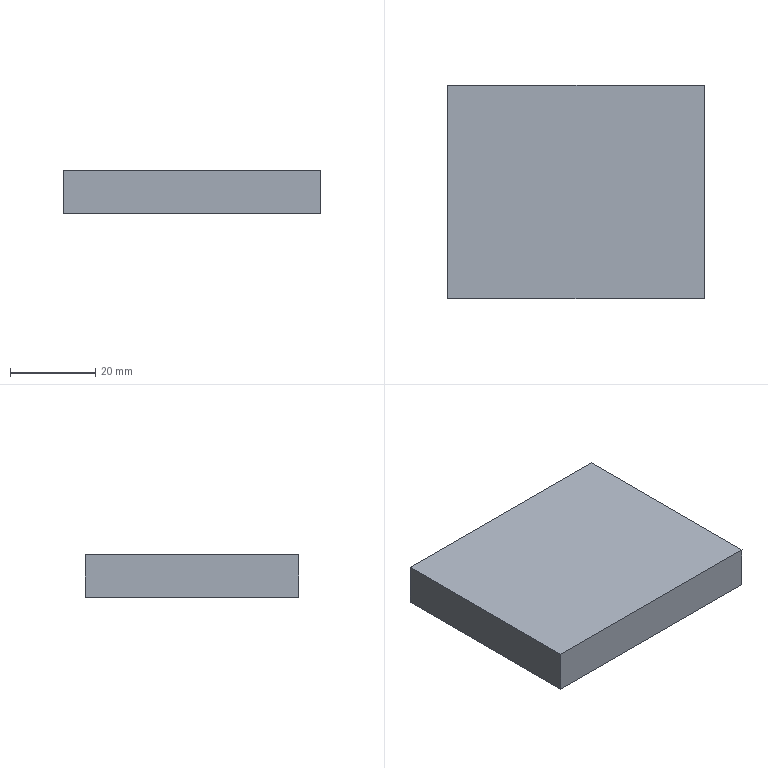Component | SolidWorks | 02-1 | 1 solid | 12 faces | box 60 x 50 x 10 mm | volume 29478 mm3 | plane 8 | cylinder 4 | commonest cylinder face diameters 6.5 x2 5 x2
build123d program:
from build123d import *

# Parameters (mm, degrees)
SKETCH1_2_W               = 60
SKETCH1_2_H               = 50
BOSS_EXTRUDE1_DEPTH       = 5
SKETCH1_R                 = 2.5
M5_TAP_CDJ2B_RODEND_DEPTH = 8
SKETCH2_R                 = 3.25
BUFFER_STOP_POCKET_DEPTH  = 11


with BuildPart() as part:
    # Sketch1_2 → Boss-Extrude1 (new, symmetric)
    with BuildSketch(Plane.XY):
        Rectangle(SKETCH1_2_W, SKETCH1_2_H)
    extrude(amount=BOSS_EXTRUDE1_DEPTH, both=True)

    # Sketch1 → M5_Tap_CDJ2B_RodEnd (cut)
    with BuildSketch(Plane.ZY.offset(30)):
        with Locations((0, -13.3)):
            Circle(SKETCH1_R)
    extrude(amount=-M5_TAP_CDJ2B_RODEND_DEPTH, mode=Mode.SUBTRACT)

    # Sketch2 → Buffer_Stop_Pocket (cut)
    with BuildSketch(Plane.ZY.offset(30)):
        with Locations((0, 11.7)):
            Circle(SKETCH2_R)
    extrude(amount=-BUFFER_STOP_POCKET_DEPTH, mode=Mode.SUBTRACT)


solid = part.part

# Placed as in the assembly
solid = solid.moved(Location((-42, 208.3, 39), (-180, 0, 180)))
STEP:
#1=CARTESIAN_POINT('',(-0.9055,8.661,1.663));
#2=VERTEX_POINT('',#1);
#3=CARTESIAN_POINT('',(-0.9055,8.661,1.407));
#4=VERTEX_POINT('',#3);
#5=CARTESIAN_POINT('',(-0.9055,8.661,1.535));
#6=DIRECTION('',(1.,0.,-0.));
#7=DIRECTION('',(0.,0.,-1.));
#8=AXIS2_PLACEMENT_3D('',#5,#6,#7);
#9=CIRCLE('',#8,0.128);
#10=EDGE_CURVE('',#2,#4,#9,.T.);
#11=ORIENTED_EDGE('',*,*,#10,.F.);
#12=CARTESIAN_POINT('',(-0.4724,8.661,1.663));
#13=VERTEX_POINT('',#12);
#14=CARTESIAN_POINT('',(-0.9055,8.661,1.663));
#15=DIRECTION('',(1.,0.,-0.));
#16=VECTOR('',#15,39.37);
#17=LINE('',#14,#16);
#18=EDGE_CURVE('',#2,#13,#17,.T.);
#19=ORIENTED_EDGE('',*,*,#18,.T.);
#20=CARTESIAN_POINT('',(-0.4724,8.661,1.407));
#21=VERTEX_POINT('',#20);
#22=CARTESIAN_POINT('',(-0.4724,8.661,1.535));
#23=DIRECTION('',(1.,0.,-0.));
#24=DIRECTION('',(0.,0.,-1.));
#25=AXIS2_PLACEMENT_3D('',#22,#23,#24);
#26=CIRCLE('',#25,0.128);
#27=EDGE_CURVE('',#13,#21,#26,.T.);
#28=ORIENTED_EDGE('',*,*,#27,.T.);
#29=CARTESIAN_POINT('',(-0.9055,8.661,1.407));
#30=DIRECTION('',(1.,0.,-0.));
#31=VECTOR('',#30,39.37);
#32=LINE('',#29,#31);
#33=EDGE_CURVE('',#4,#21,#32,.T.);
#34=ORIENTED_EDGE('',*,*,#33,.F.);
#35=EDGE_LOOP('',(#11,#19,#28,#34));
#36=FACE_OUTER_BOUND('',#35,.T.);
#37=CARTESIAN_POINT('',(-0.9055,8.661,1.535));
#38=DIRECTION('',(1.,0.,-0.));
#39=DIRECTION('',(0.,0.,-1.));
#40=AXIS2_PLACEMENT_3D('',#37,#38,#39);
#41=CYLINDRICAL_SURFACE('',#40,0.128);
#42=ADVANCED_FACE('',(#36),#41,.F.);
#43=CARTESIAN_POINT('',(-0.7874,7.677,1.634));
#44=VERTEX_POINT('',#43);
#45=CARTESIAN_POINT('',(-0.7874,7.677,1.437));
#46=VERTEX_POINT('',#45);
#47=CARTESIAN_POINT('',(-0.7874,7.677,1.535));
#48=DIRECTION('',(1.,0.,-0.));
#49=DIRECTION('',(0.,0.,-1.));
#50=AXIS2_PLACEMENT_3D('',#47,#48,#49);
#51=CIRCLE('',#50,0.09843);
#52=EDGE_CURVE('',#44,#46,#51,.T.);
#53=ORIENTED_EDGE('',*,*,#52,.F.);
#54=CARTESIAN_POINT('',(-0.4724,7.677,1.634));
#55=VERTEX_POINT('',#54);
#56=CARTESIAN_POINT('',(-0.7874,7.677,1.634));
#57=DIRECTION('',(1.,0.,-0.));
#58=VECTOR('',#57,39.37);
#59=LINE('',#56,#58);
#60=EDGE_CURVE('',#44,#55,#59,.T.);
#61=ORIENTED_EDGE('',*,*,#60,.T.);
#62=CARTESIAN_POINT('',(-0.4724,7.677,1.437));
#63=VERTEX_POINT('',#62);
#64=CARTESIAN_POINT('',(-0.4724,7.677,1.535));
#65=DIRECTION('',(1.,0.,-0.));
#66=DIRECTION('',(0.,0.,-1.));
#67=AXIS2_PLACEMENT_3D('',#64,#65,#66);
#68=CIRCLE('',#67,0.09843);
#69=EDGE_CURVE('',#55,#63,#68,.T.);
#70=ORIENTED_EDGE('',*,*,#69,.T.);
#71=CARTESIAN_POINT('',(-0.7874,7.677,1.437));
#72=DIRECTION('',(1.,0.,-0.));
#73=VECTOR('',#72,39.37);
#74=LINE('',#71,#73);
#75=EDGE_CURVE('',#46,#63,#74,.T.);
#76=ORIENTED_EDGE('',*,*,#75,.F.);
#77=EDGE_LOOP('',(#53,#61,#70,#76));
#78=FACE_OUTER_BOUND('',#77,.T.);
#79=CARTESIAN_POINT('',(-0.7874,7.677,1.535));
#80=DIRECTION('',(1.,0.,-0.));
#81=DIRECTION('',(0.,0.,-1.));
#82=AXIS2_PLACEMENT_3D('',#79,#80,#81);
#83=CYLINDRICAL_SURFACE('',#82,0.09843);
#84=ADVANCED_FACE('',(#78),#83,.F.);
#85=CARTESIAN_POINT('',(-2.835,7.217,1.732));
#86=VERTEX_POINT('',#85);
#87=CARTESIAN_POINT('',(-2.835,9.185,1.732));
#88=VERTEX_POINT('',#87);
#89=CARTESIAN_POINT('',(-2.835,7.217,1.732));
#90=DIRECTION('',(-0.,1.,0.));
#91=VECTOR('',#90,39.37);
#92=LINE('',#89,#91);
#93=EDGE_CURVE('',#86,#88,#92,.T.);
#94=ORIENTED_EDGE('',*,*,#93,.T.);
#95=CARTESIAN_POINT('',(-2.835,9.185,1.339));
#96=VERTEX_POINT('',#95);
#97=CARTESIAN_POINT('',(-2.835,9.185,1.339));
#98=DIRECTION('',(0.,-0.,1.));
#99=VECTOR('',#98,39.37);
#100=LINE('',#97,#99);
#101=EDGE_CURVE('',#96,#88,#100,.T.);
#102=ORIENTED_EDGE('',*,*,#101,.F.);
#103=CARTESIAN_POINT('',(-2.835,7.217,1.339));
#104=VERTEX_POINT('',#103);
#105=CARTESIAN_POINT('',(-2.835,7.217,1.339));
#106=DIRECTION('',(-0.,1.,0.));
#107=VECTOR('',#106,39.37);
#108=LINE('',#105,#107);
#109=EDGE_CURVE('',#104,#96,#108,.T.);
#110=ORIENTED_EDGE('',*,*,#109,.F.);
#111=CARTESIAN_POINT('',(-2.835,7.217,1.339));
#112=DIRECTION('',(0.,-0.,1.));
#113=VECTOR('',#112,39.37);
#114=LINE('',#111,#113);
#115=EDGE_CURVE('',#104,#86,#114,.T.);
#116=ORIENTED_EDGE('',*,*,#115,.T.);
#117=EDGE_LOOP('',(#94,#102,#110,#116));
#118=FACE_OUTER_BOUND('',#117,.T.);
#119=CARTESIAN_POINT('',(-2.835,7.217,1.339));
#120=DIRECTION('',(1.,0.,-0.));
#121=DIRECTION('',(-0.,0.,-1.));
#122=AXIS2_PLACEMENT_3D('',#119,#120,#121);
#123=PLANE('',#122);
#124=ADVANCED_FACE('',(#118),#123,.F.);
#125=CARTESIAN_POINT('',(-0.4724,9.185,1.732));
#126=VERTEX_POINT('',#125);
#127=CARTESIAN_POINT('',(-0.4724,9.185,1.732));
#128=DIRECTION('',(1.,0.,-0.));
#129=VECTOR('',#128,39.37);
#130=LINE('',#127,#129);
#131=EDGE_CURVE('',#88,#126,#130,.T.);
#132=ORIENTED_EDGE('',*,*,#131,.T.);
#133=CARTESIAN_POINT('',(-0.4724,9.185,1.339));
#134=VERTEX_POINT('',#133);
#135=CARTESIAN_POINT('',(-0.4724,9.185,1.339));
#136=DIRECTION('',(0.,-0.,1.));
#137=VECTOR('',#136,39.37);
#138=LINE('',#135,#137);
#139=EDGE_CURVE('',#134,#126,#138,.T.);
#140=ORIENTED_EDGE('',*,*,#139,.F.);
#141=CARTESIAN_POINT('',(-0.4724,9.185,1.339));
#142=DIRECTION('',(1.,0.,-0.));
#143=VECTOR('',#142,39.37);
#144=LINE('',#141,#143);
#145=EDGE_CURVE('',#96,#134,#144,.T.);
#146=ORIENTED_EDGE('',*,*,#145,.F.);
#147=ORIENTED_EDGE('',*,*,#101,.T.);
#148=EDGE_LOOP('',(#132,#140,#146,#147));
#149=FACE_OUTER_BOUND('',#148,.T.);
#150=CARTESIAN_POINT('',(-0.4724,9.185,1.339));
#151=DIRECTION('',(0.,-1.,-0.));
#152=DIRECTION('',(0.,-0.,1.));
#153=AXIS2_PLACEMENT_3D('',#150,#151,#152);
#154=PLANE('',#153);
#155=ADVANCED_FACE('',(#149),#154,.F.);
#156=CARTESIAN_POINT('',(-0.4724,8.661,1.535));
#157=DIRECTION('',(1.,0.,-0.));
#158=DIRECTION('',(0.,0.,-1.));
#159=AXIS2_PLACEMENT_3D('',#156,#157,#158);
#160=CIRCLE('',#159,0.128);
#161=EDGE_CURVE('',#21,#13,#160,.T.);
#162=ORIENTED_EDGE('',*,*,#161,.F.);
#163=ORIENTED_EDGE('',*,*,#27,.F.);
#164=EDGE_LOOP('',(#162,#163));
#165=FACE_BOUND('',#164,.T.);
#166=CARTESIAN_POINT('',(-0.4724,7.677,1.535));
#167=DIRECTION('',(1.,0.,-0.));
#168=DIRECTION('',(0.,0.,-1.));
#169=AXIS2_PLACEMENT_3D('',#166,#167,#168);
#170=CIRCLE('',#169,0.09843);
#171=EDGE_CURVE('',#63,#55,#170,.T.);
#172=ORIENTED_EDGE('',*,*,#171,.F.);
#173=ORIENTED_EDGE('',*,*,#69,.F.);
#174=EDGE_LOOP('',(#172,#173));
#175=FACE_BOUND('',#174,.T.);
#176=CARTESIAN_POINT('',(-0.4724,7.217,1.732));
#177=VERTEX_POINT('',#176);
#178=CARTESIAN_POINT('',(-0.4724,7.217,1.732));
#179=DIRECTION('',(0.,-1.,-0.));
#180=VECTOR('',#179,39.37);
#181=LINE('',#178,#180);
#182=EDGE_CURVE('',#126,#177,#181,.T.);
#183=ORIENTED_EDGE('',*,*,#182,.T.);
#184=CARTESIAN_POINT('',(-0.4724,7.217,1.339));
#185=VERTEX_POINT('',#184);
#186=CARTESIAN_POINT('',(-0.4724,7.217,1.339));
#187=DIRECTION('',(0.,-0.,1.));
#188=VECTOR('',#187,39.37);
#189=LINE('',#186,#188);
#190=EDGE_CURVE('',#185,#177,#189,.T.);
#191=ORIENTED_EDGE('',*,*,#190,.F.);
#192=CARTESIAN_POINT('',(-0.4724,7.217,1.339));
#193=DIRECTION('',(0.,-1.,-0.));
#194=VECTOR('',#193,39.37);
#195=LINE('',#192,#194);
#196=EDGE_CURVE('',#134,#185,#195,.T.);
#197=ORIENTED_EDGE('',*,*,#196,.F.);
#198=ORIENTED_EDGE('',*,*,#139,.T.);
#199=EDGE_LOOP('',(#183,#191,#197,#198));
#200=FACE_OUTER_BOUND('',#199,.T.);
#201=CARTESIAN_POINT('',(-0.4724,7.217,1.339));
#202=DIRECTION('',(-1.,-0.,0.));
#203=DIRECTION('',(0.,-0.,1.));
#204=AXIS2_PLACEMENT_3D('',#201,#202,#203);
#205=PLANE('',#204);
#206=ADVANCED_FACE('',(#165,#175,#200),#205,.F.);
#207=CARTESIAN_POINT('',(-0.4724,7.217,1.732));
#208=DIRECTION('',(-1.,-0.,0.));
#209=VECTOR('',#208,39.37);
#210=LINE('',#207,#209);
#211=EDGE_CURVE('',#177,#86,#210,.T.);
#212=ORIENTED_EDGE('',*,*,#211,.T.);
#213=ORIENTED_EDGE('',*,*,#115,.F.);
#214=CARTESIAN_POINT('',(-0.4724,7.217,1.339));
#215=DIRECTION('',(-1.,-0.,0.));
#216=VECTOR('',#215,39.37);
#217=LINE('',#214,#216);
#218=EDGE_CURVE('',#185,#104,#217,.T.);
#219=ORIENTED_EDGE('',*,*,#218,.F.);
#220=ORIENTED_EDGE('',*,*,#190,.T.);
#221=EDGE_LOOP('',(#212,#213,#219,#220));
#222=FACE_OUTER_BOUND('',#221,.T.);
#223=CARTESIAN_POINT('',(-0.4724,7.217,1.339));
#224=DIRECTION('',(-0.,1.,0.));
#225=DIRECTION('',(-0.,0.,-1.));
#226=AXIS2_PLACEMENT_3D('',#223,#224,#225);
#227=PLANE('',#226);
#228=ADVANCED_FACE('',(#222),#227,.F.);
#229=ORIENTED_EDGE('',*,*,#109,.T.);
#230=ORIENTED_EDGE('',*,*,#145,.T.);
#231=ORIENTED_EDGE('',*,*,#196,.T.);
#232=ORIENTED_EDGE('',*,*,#218,.T.);
#233=EDGE_LOOP('',(#229,#230,#231,#232));
#234=FACE_OUTER_BOUND('',#233,.T.);
#235=CARTESIAN_POINT('',(-1.654,8.201,1.339));
#236=DIRECTION('',(0.,-0.,1.));
#237=DIRECTION('',(1.,0.,-0.));
#238=AXIS2_PLACEMENT_3D('',#235,#236,#237);
#239=PLANE('',#238);
#240=ADVANCED_FACE('',(#234),#239,.F.);
#241=ORIENTED_EDGE('',*,*,#93,.F.);
#242=ORIENTED_EDGE('',*,*,#211,.F.);
#243=ORIENTED_EDGE('',*,*,#182,.F.);
#244=ORIENTED_EDGE('',*,*,#131,.F.);
#245=EDGE_LOOP('',(#241,#242,#243,#244));
#246=FACE_OUTER_BOUND('',#245,.T.);
#247=CARTESIAN_POINT('',(-1.654,8.201,1.732));
#248=DIRECTION('',(0.,-0.,1.));
#249=DIRECTION('',(1.,0.,-0.));
#250=AXIS2_PLACEMENT_3D('',#247,#248,#249);
#251=PLANE('',#250);
#252=ADVANCED_FACE('',(#246),#251,.T.);
#253=ORIENTED_EDGE('',*,*,#60,.F.);
#254=CARTESIAN_POINT('',(-0.7874,7.677,1.535));
#255=DIRECTION('',(1.,0.,-0.));
#256=DIRECTION('',(0.,0.,-1.));
#257=AXIS2_PLACEMENT_3D('',#254,#255,#256);
#258=CIRCLE('',#257,0.09843);
#259=EDGE_CURVE('',#46,#44,#258,.T.);
#260=ORIENTED_EDGE('',*,*,#259,.F.);
#261=ORIENTED_EDGE('',*,*,#75,.T.);
#262=ORIENTED_EDGE('',*,*,#171,.T.);
#263=EDGE_LOOP('',(#253,#260,#261,#262));
#264=FACE_OUTER_BOUND('',#263,.T.);
#265=CARTESIAN_POINT('',(-0.7874,7.677,1.535));
#266=DIRECTION('',(1.,0.,-0.));
#267=DIRECTION('',(0.,0.,-1.));
#268=AXIS2_PLACEMENT_3D('',#265,#266,#267);
#269=CYLINDRICAL_SURFACE('',#268,0.09843);
#270=ADVANCED_FACE('',(#264),#269,.F.);
#271=ORIENTED_EDGE('',*,*,#259,.T.);
#272=ORIENTED_EDGE('',*,*,#52,.T.);
#273=EDGE_LOOP('',(#271,#272));
#274=FACE_OUTER_BOUND('',#273,.T.);
#275=CARTESIAN_POINT('',(-0.7874,7.677,1.535));
#276=DIRECTION('',(1.,0.,-0.));
#277=DIRECTION('',(-0.,0.,-1.));
#278=AXIS2_PLACEMENT_3D('',#275,#276,#277);
#279=PLANE('',#278);
#280=ADVANCED_FACE('',(#274),#279,.T.);
#281=ORIENTED_EDGE('',*,*,#18,.F.);
#282=CARTESIAN_POINT('',(-0.9055,8.661,1.535));
#283=DIRECTION('',(1.,0.,-0.));
#284=DIRECTION('',(0.,0.,-1.));
#285=AXIS2_PLACEMENT_3D('',#282,#283,#284);
#286=CIRCLE('',#285,0.128);
#287=EDGE_CURVE('',#4,#2,#286,.T.);
#288=ORIENTED_EDGE('',*,*,#287,.F.);
#289=ORIENTED_EDGE('',*,*,#33,.T.);
#290=ORIENTED_EDGE('',*,*,#161,.T.);
#291=EDGE_LOOP('',(#281,#288,#289,#290));
#292=FACE_OUTER_BOUND('',#291,.T.);
#293=CARTESIAN_POINT('',(-0.9055,8.661,1.535));
#294=DIRECTION('',(1.,0.,-0.));
#295=DIRECTION('',(0.,0.,-1.));
#296=AXIS2_PLACEMENT_3D('',#293,#294,#295);
#297=CYLINDRICAL_SURFACE('',#296,0.128);
#298=ADVANCED_FACE('',(#292),#297,.F.);
#299=ORIENTED_EDGE('',*,*,#287,.T.);
#300=ORIENTED_EDGE('',*,*,#10,.T.);
#301=EDGE_LOOP('',(#299,#300));
#302=FACE_OUTER_BOUND('',#301,.T.);
#303=CARTESIAN_POINT('',(-0.9055,8.661,1.535));
#304=DIRECTION('',(1.,0.,-0.));
#305=DIRECTION('',(-0.,0.,-1.));
#306=AXIS2_PLACEMENT_3D('',#303,#304,#305);
#307=PLANE('',#306);
#308=ADVANCED_FACE('',(#302),#307,.T.);
#309=CLOSED_SHELL('',(#42,#84,#124,#155,#206,#228,#240,#252,#270,#280,#298,#308));
#310=MANIFOLD_SOLID_BREP('',#309);
#311=CARTESIAN_POINT('',(0.,0.,0.));
#312=DIRECTION('',(0.,0.,1.));
#313=DIRECTION('',(1.,0.,0.));
#314=AXIS2_PLACEMENT_3D('',#311,#312,#313);
#315=(LENGTH_UNIT()NAMED_UNIT(*)SI_UNIT($,.METRE.));
#316=LENGTH_MEASURE_WITH_UNIT(LENGTH_MEASURE(0.0254),#315);
#317=DIMENSIONAL_EXPONENTS(1.,0.,0.,0.,0.,0.,0.);
#318=(CONVERSION_BASED_UNIT('',#316)LENGTH_UNIT()NAMED_UNIT(#317));
#319=UNCERTAINTY_MEASURE_WITH_UNIT(LENGTH_MEASURE(0.00001),#318,'','');
#320=(NAMED_UNIT(*)PLANE_ANGLE_UNIT()SI_UNIT($,.RADIAN.));
#321=(NAMED_UNIT(*)SI_UNIT($,.STERADIAN.)SOLID_ANGLE_UNIT());
#322=(GEOMETRIC_REPRESENTATION_CONTEXT(3)GLOBAL_UNCERTAINTY_ASSIGNED_CONTEXT((#319))GLOBAL_UNIT_ASSIGNED_CONTEXT((#318,#320,#321))REPRESENTATION_CONTEXT('',''));
#323=ADVANCED_BREP_SHAPE_REPRESENTATION('',(#310,#314),#322);
#324=COLOUR_RGB('',0.7922,0.8196,0.9333);
#325=FILL_AREA_STYLE_COLOUR('',#324);
#326=FILL_AREA_STYLE('',(#325));
#327=SURFACE_STYLE_FILL_AREA(#326);
#328=SURFACE_SIDE_STYLE('',(#327));
#329=SURFACE_STYLE_USAGE(.BOTH.,#328);
#330=PRESENTATION_STYLE_ASSIGNMENT((#329));
#331=STYLED_ITEM('',(#330),#310);
#332=(LENGTH_UNIT()NAMED_UNIT(*)SI_UNIT($,.METRE.));
#333=LENGTH_MEASURE_WITH_UNIT(LENGTH_MEASURE(0.0254),#332);
#334=DIMENSIONAL_EXPONENTS(1.,0.,0.,0.,0.,0.,0.);
#335=(CONVERSION_BASED_UNIT('',#333)LENGTH_UNIT()NAMED_UNIT(#334));
#336=UNCERTAINTY_MEASURE_WITH_UNIT(LENGTH_MEASURE(0.00001),#335,'','');
#337=(NAMED_UNIT(*)PLANE_ANGLE_UNIT()SI_UNIT($,.RADIAN.));
#338=(NAMED_UNIT(*)SI_UNIT($,.STERADIAN.)SOLID_ANGLE_UNIT());
#339=(GEOMETRIC_REPRESENTATION_CONTEXT(3)GLOBAL_UNCERTAINTY_ASSIGNED_CONTEXT((#336))GLOBAL_UNIT_ASSIGNED_CONTEXT((#335,#337,#338))REPRESENTATION_CONTEXT('',''));
#340=MECHANICAL_DESIGN_GEOMETRIC_PRESENTATION_REPRESENTATION('',(#331),#339);
#341=PRESENTATION_LAYER_ASSIGNMENT('','',(#331));